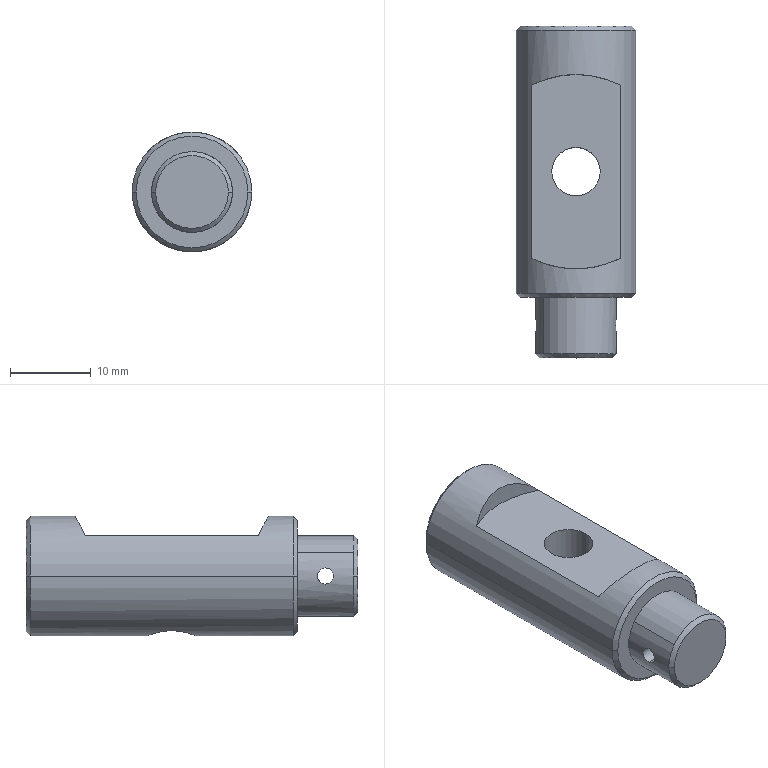CAM job | Mastercam | mm | 7 operations | part box 14.8 x 41 x 14.8
1. 2D High Speed (2D Blend Mill) | 8 - 8 平铣刀
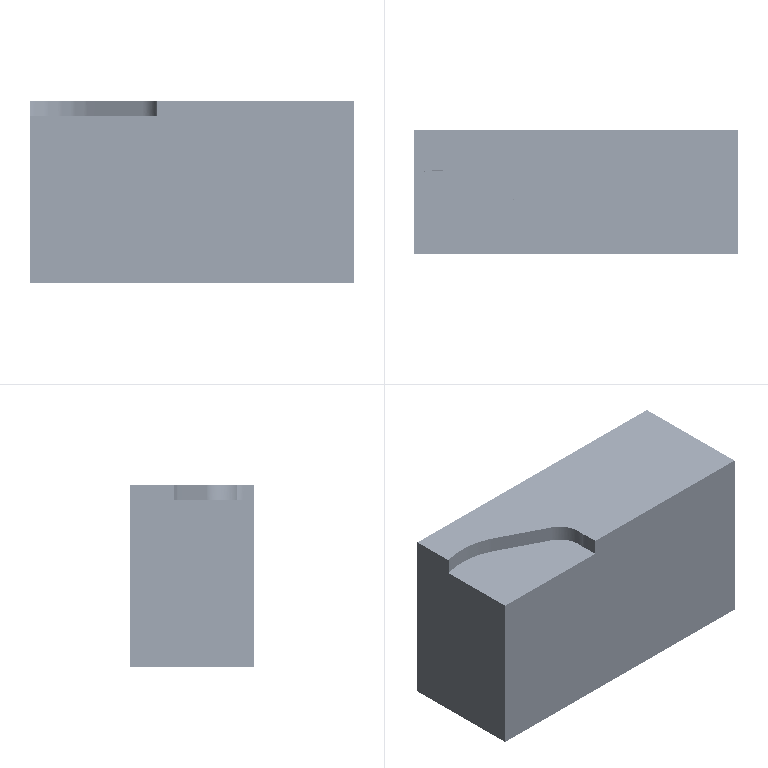2. 2D High Speed (2D Blend Mill) | 9 - 8 平铣刀
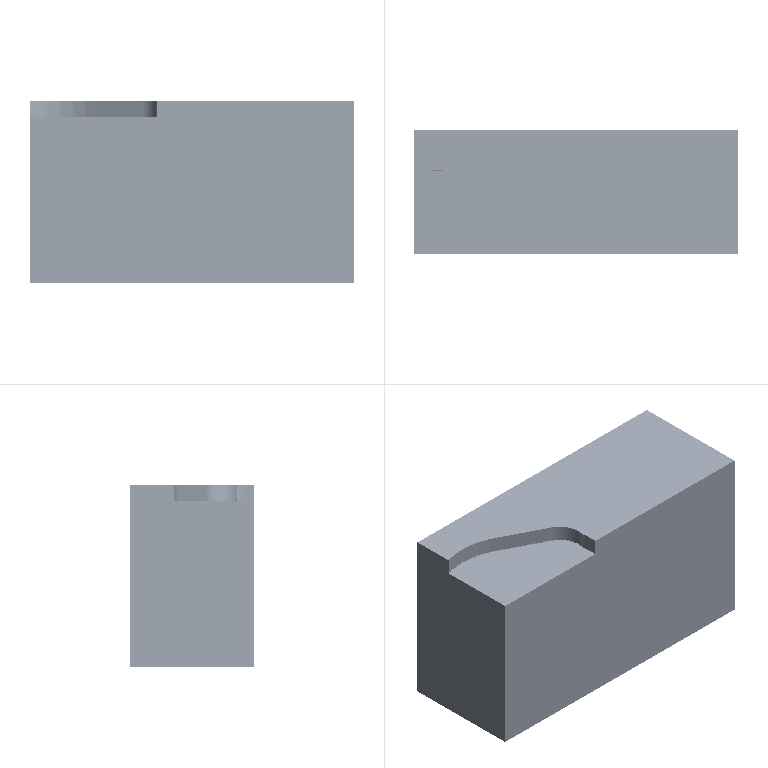3. Contour (2D) | 9 - 8 平铣刀
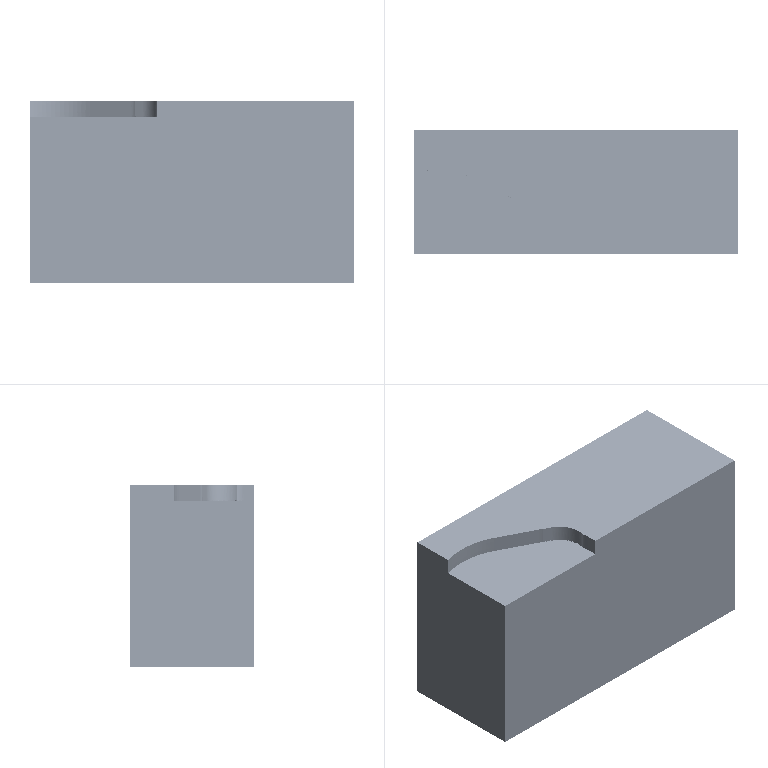4. Drill/Counterbore | 7 - 4 倒角刀
5. Peck Drill | 1 - 5.1 钻头
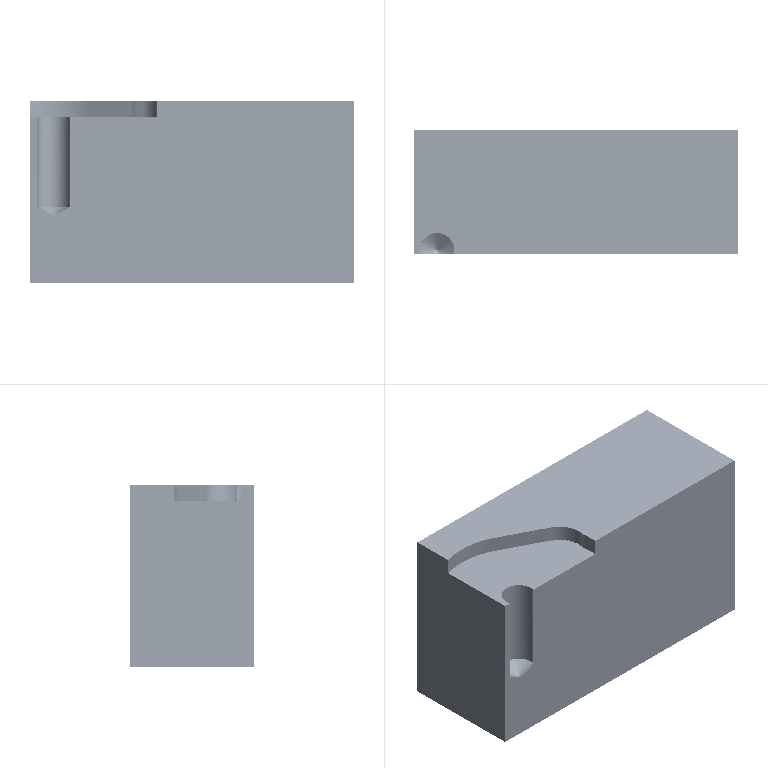6. Drill/Counterbore | 7 - 4 倒角刀
7. Peck Drill | 18 - 2 钻头